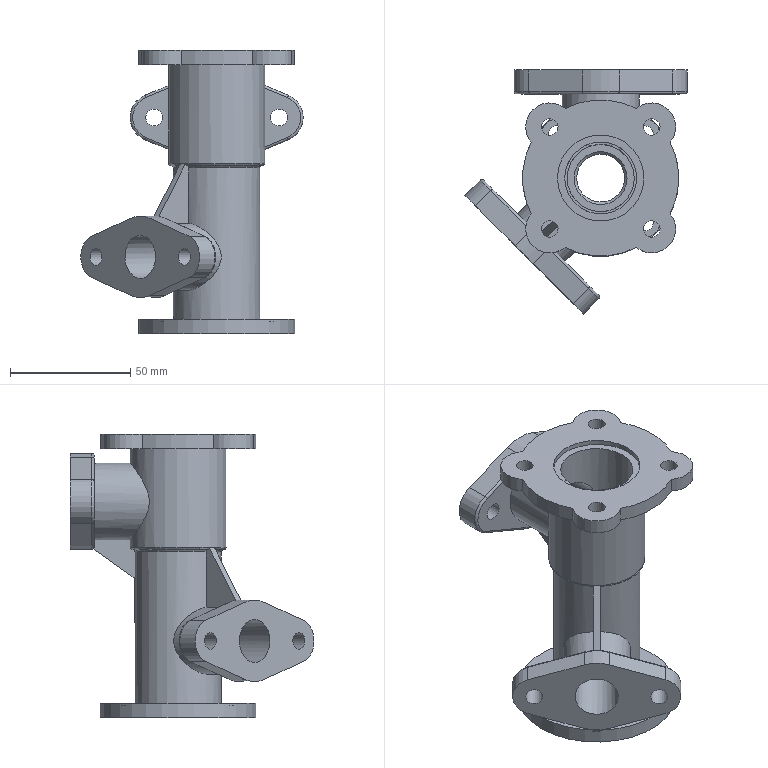Component | NX | LOWER_VALVE_BODY | 1 solid | 102 faces | volume 130238 mm3 | cylinder 56 | plane 34 | torus 11 | cone 1 | commonest cylinder face diameters 7 x12 2 x8 20 x7 65 x5 13 x4 12.5 x4 40 x3 18 x3